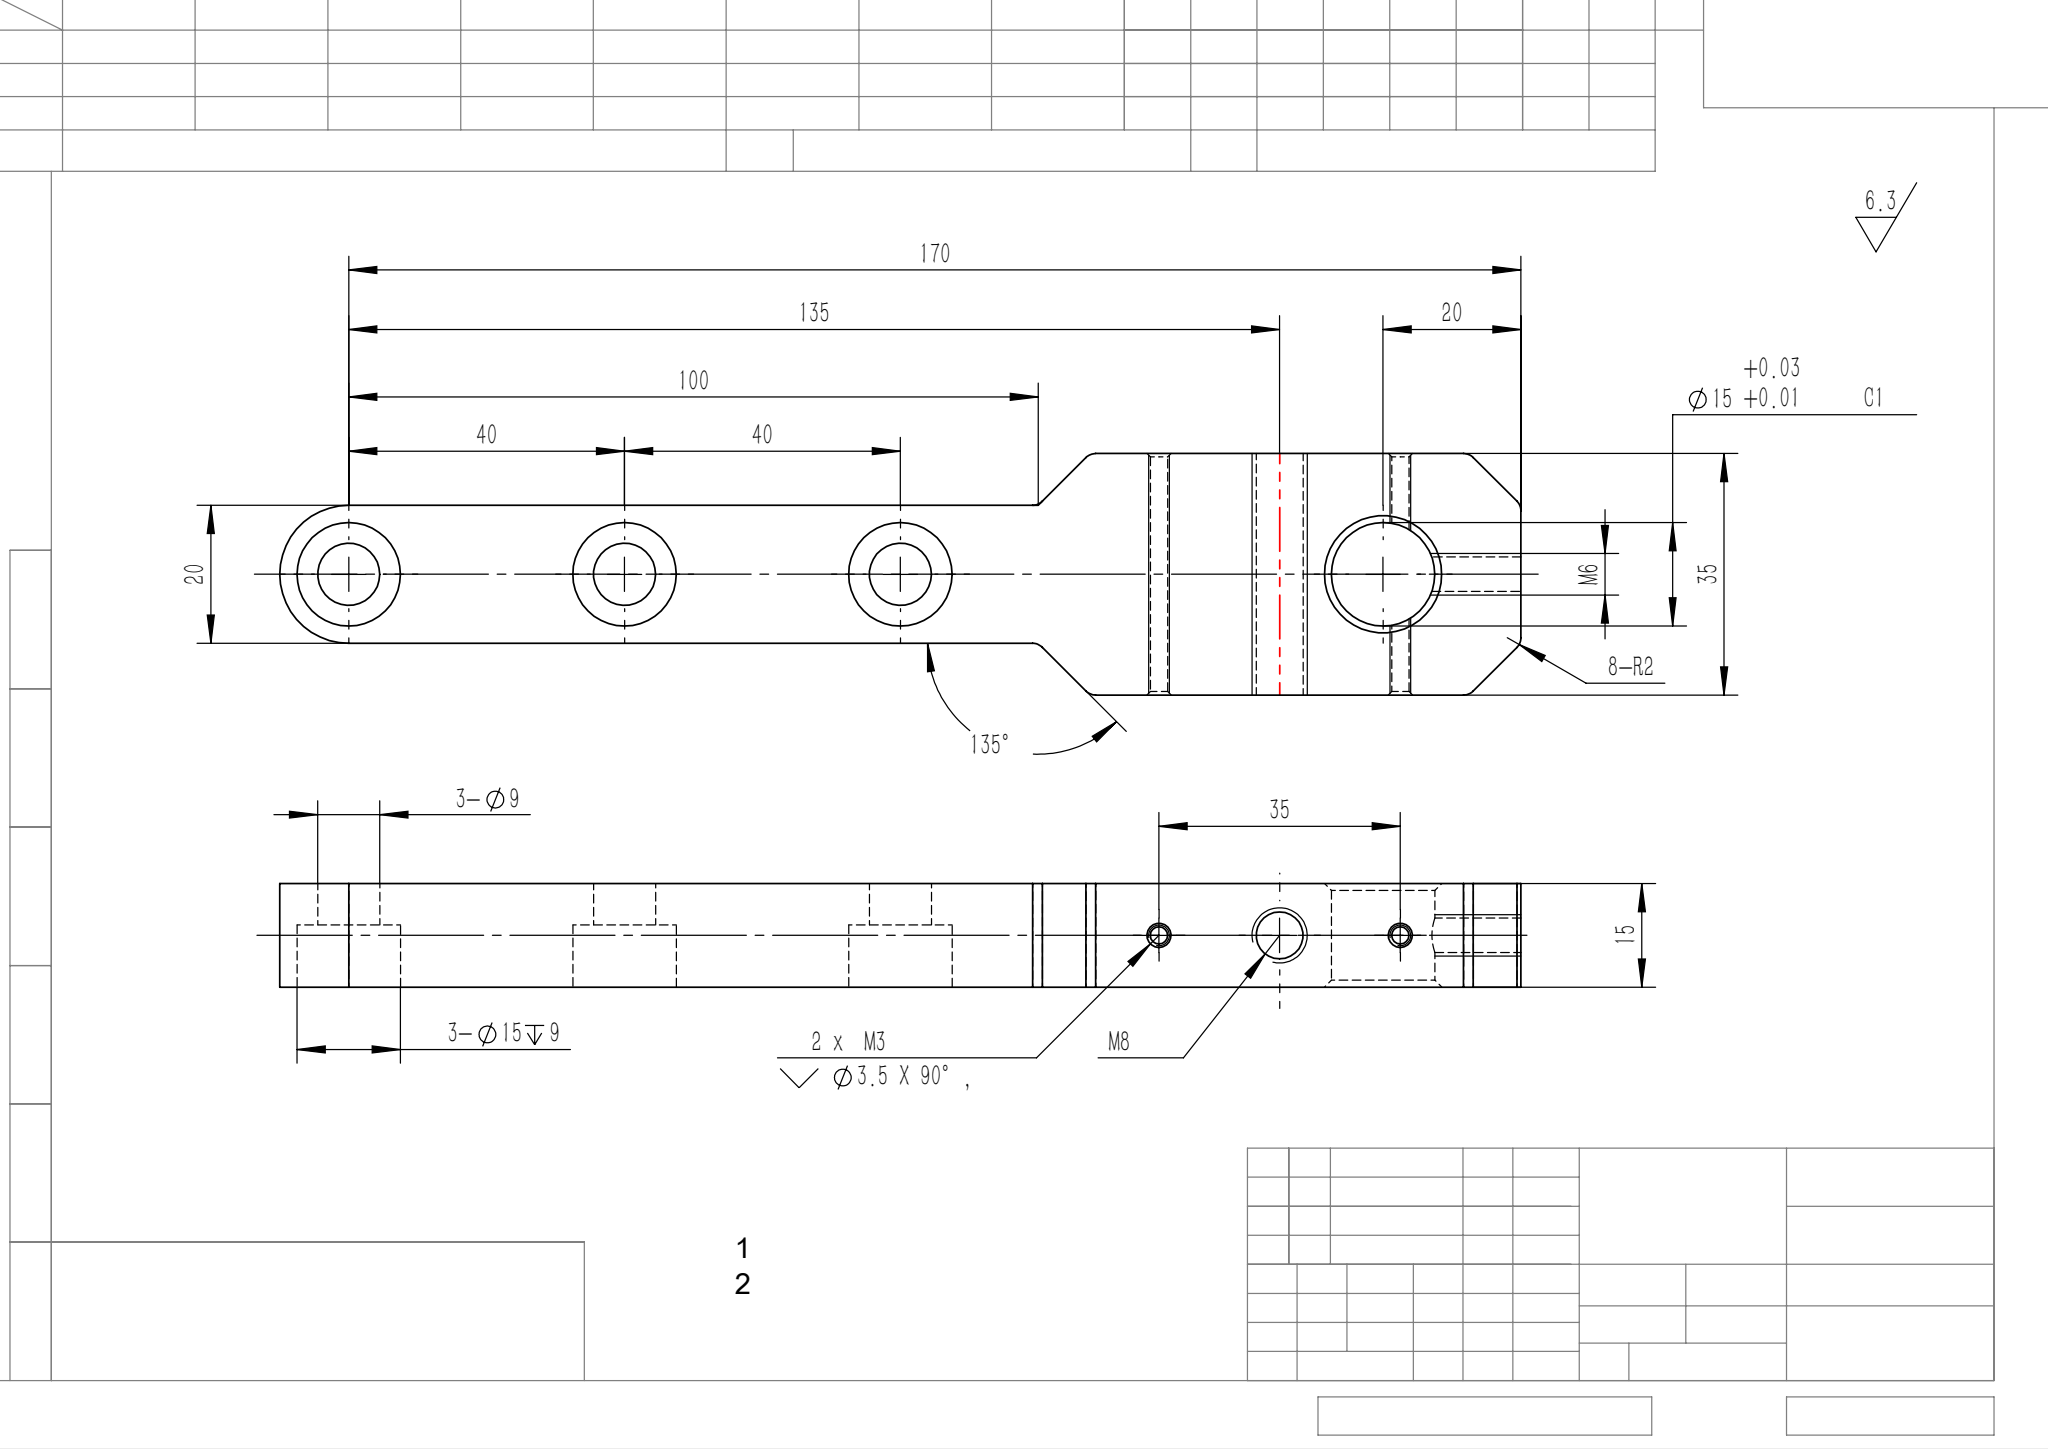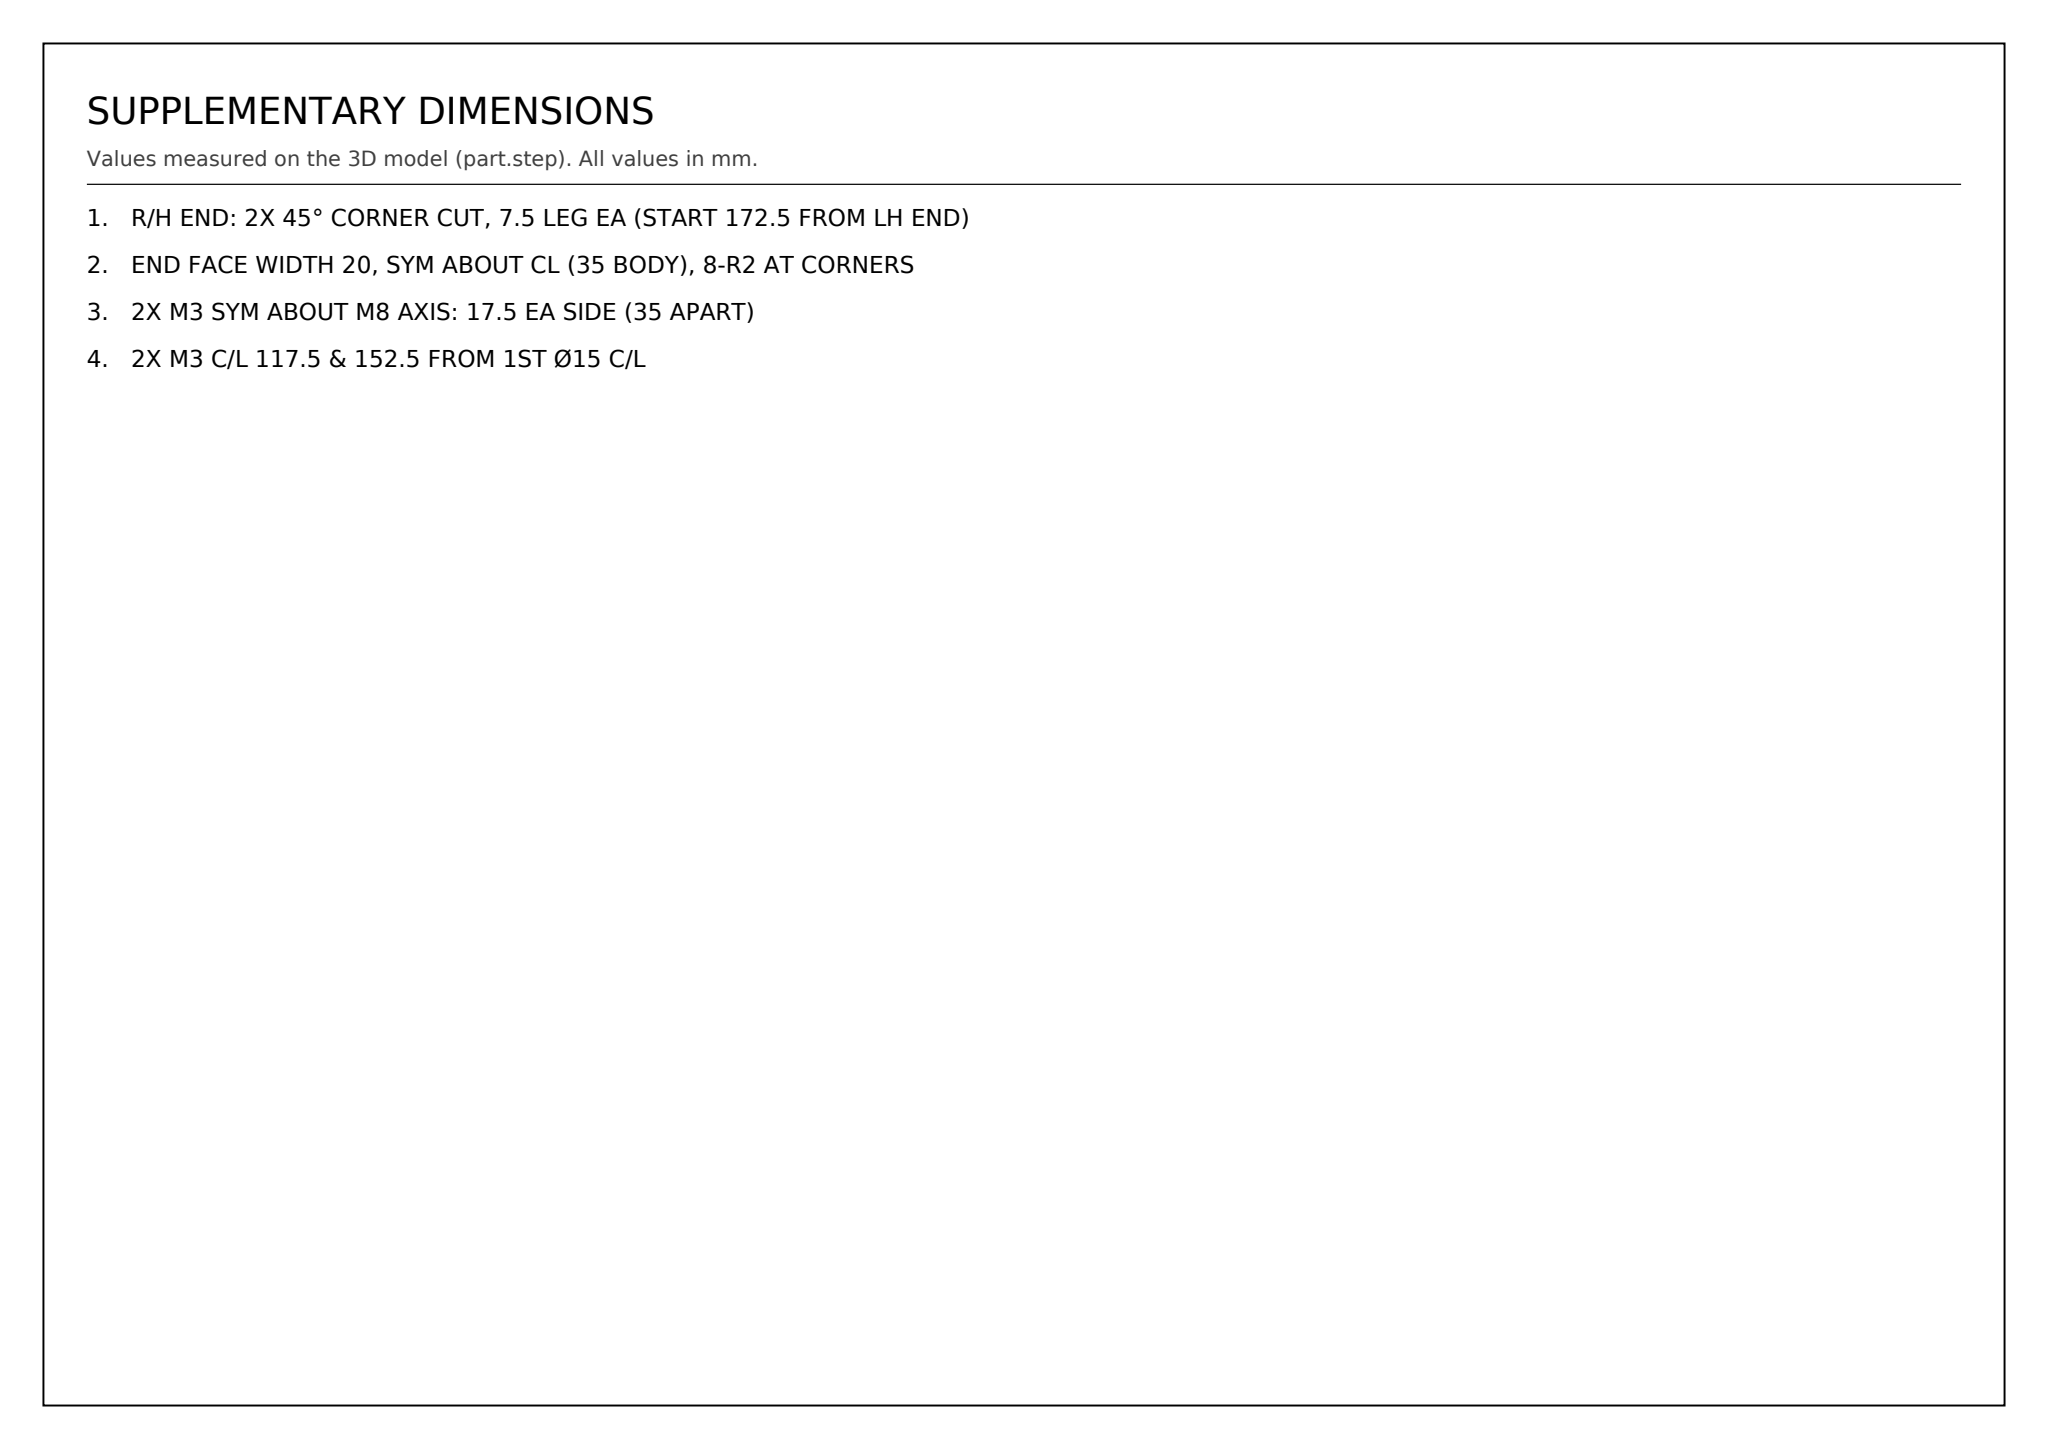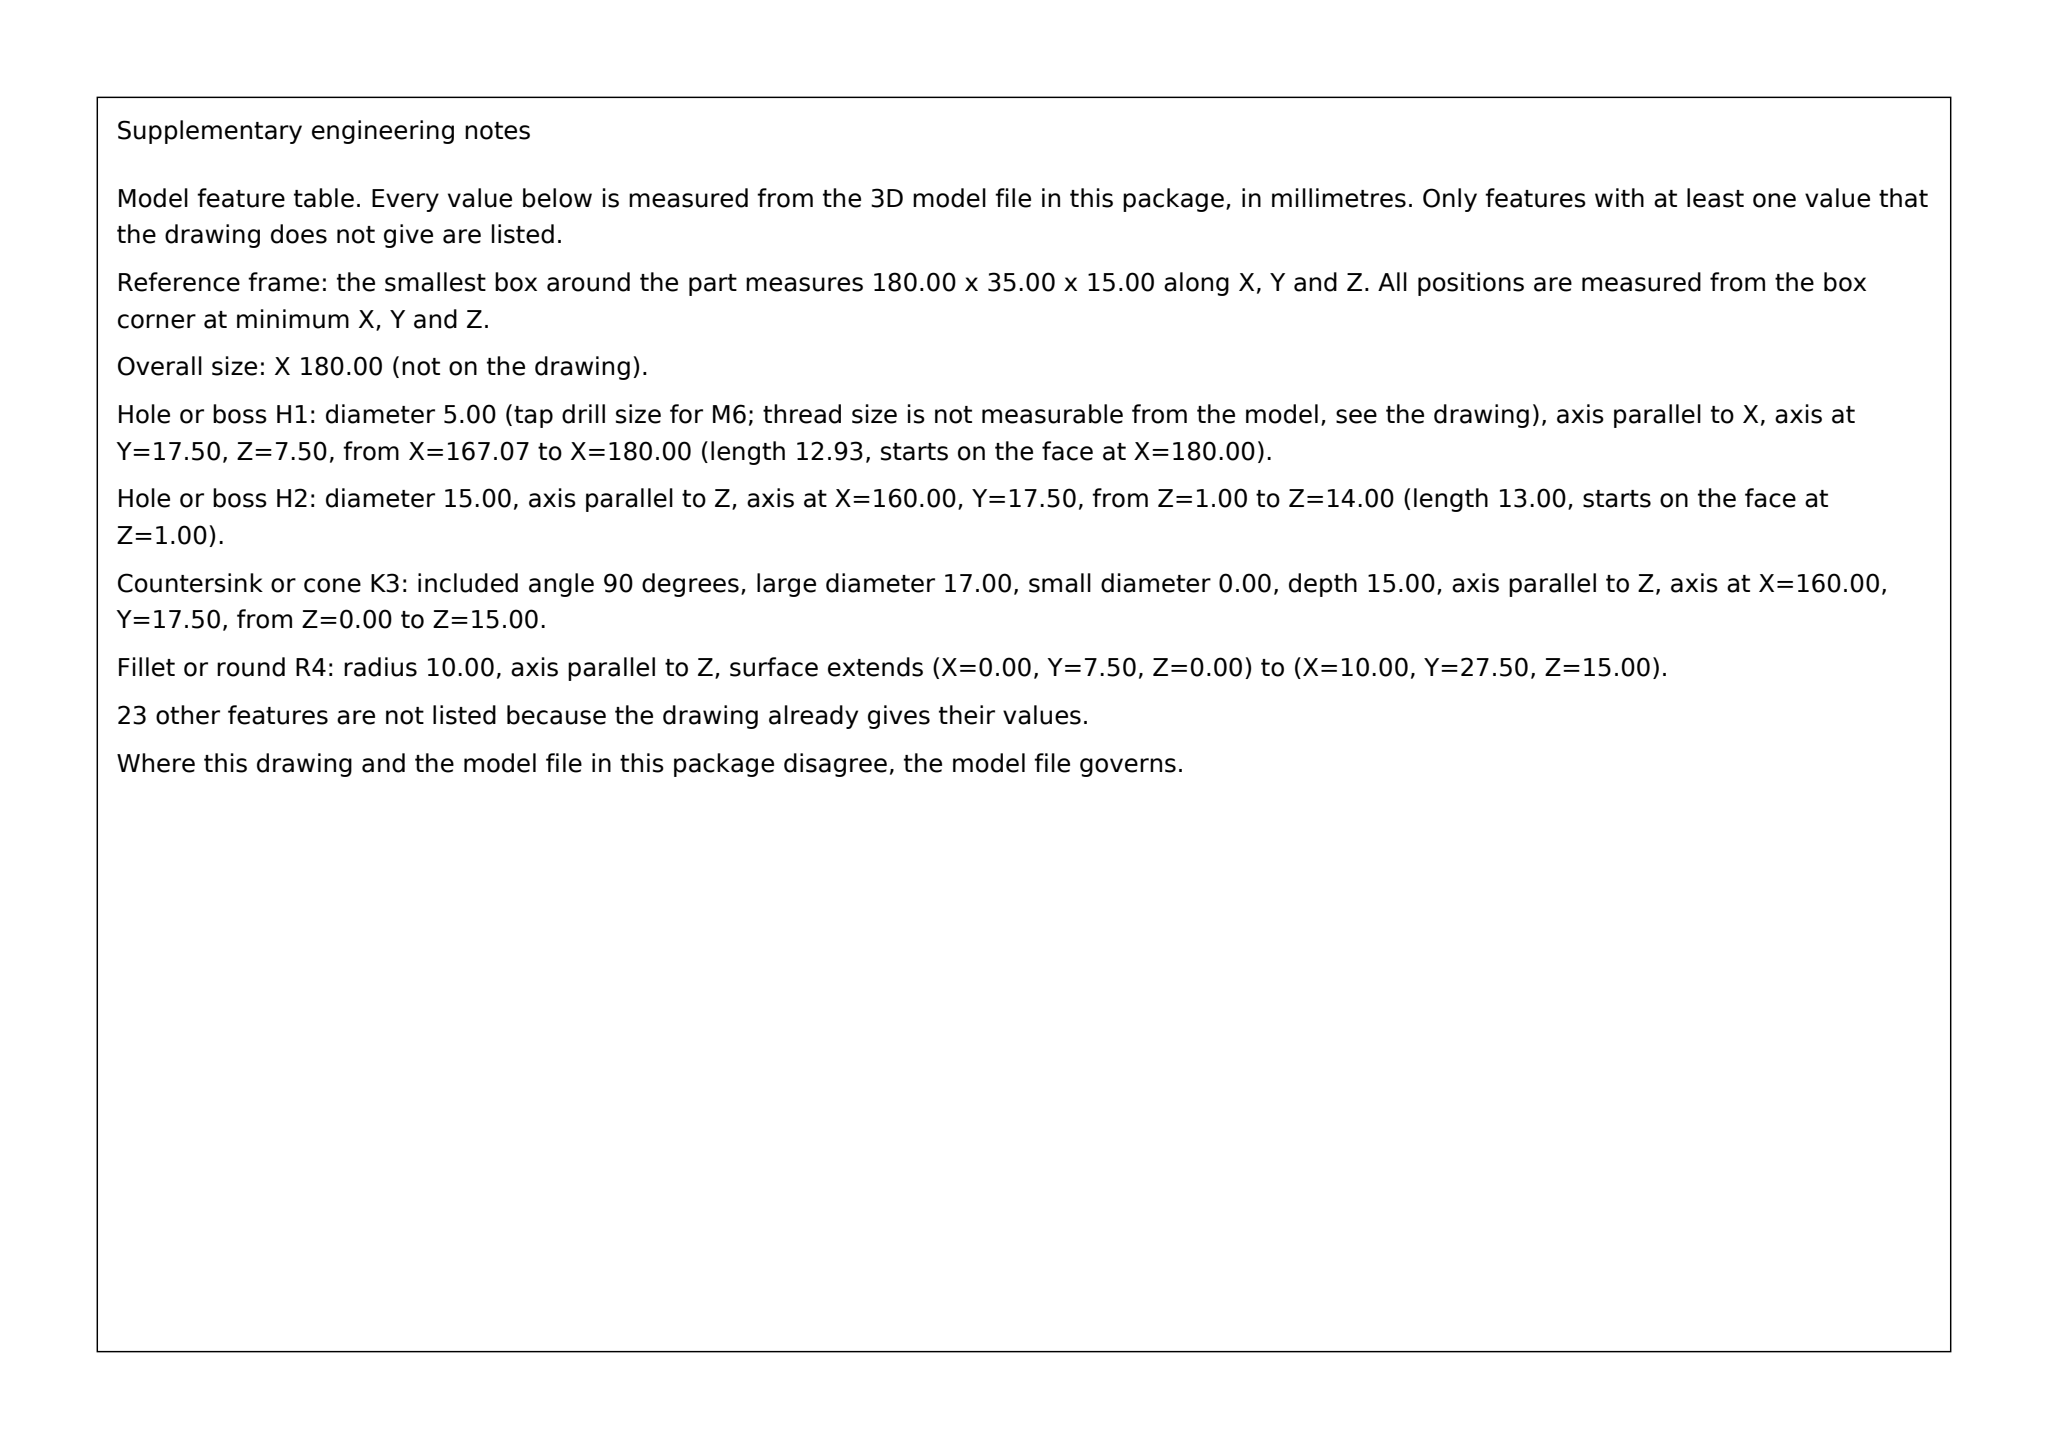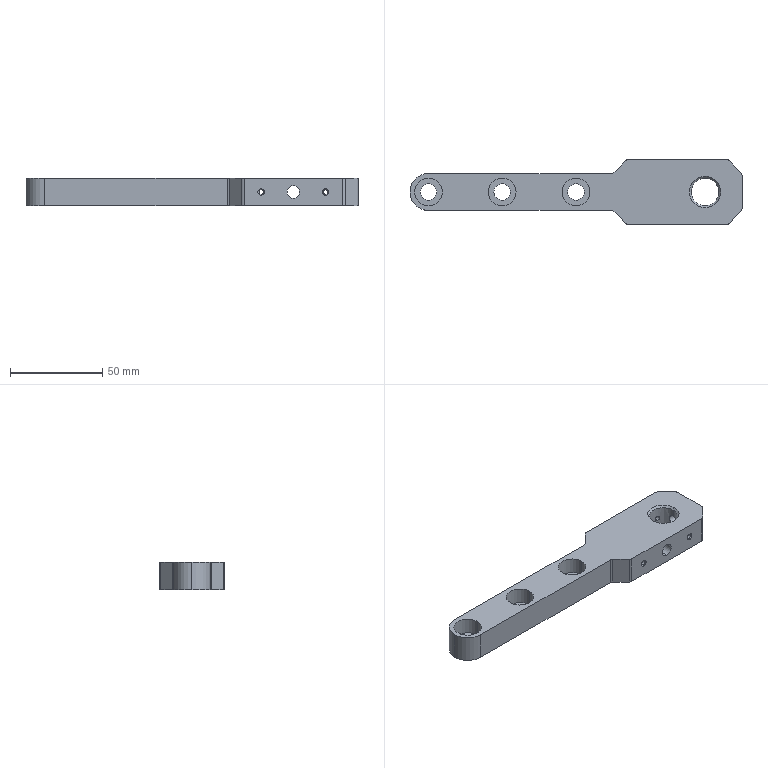Part | SolidWorks | mm | 1 solid | 60 faces | box 180 x 35 x 15 mm | volume 57000 mm3 | cylinder 34 | plane 14 | cone 12 | commonest cylinder face diameters 15 x8 4 x8 2.5 x6 9 x6 6.8 x2 5 x2 20 x2
Drawing notes:
R/H END: 2X 45° CORNER CUT, 7.5 LEG EA (START 172.5 FROM LH END) | from the solid: End face plane x=180 with y-planes 7.5 & 27.5; R2 fillet centers (171.67,33) & (178,8.33) fit 45° line x+y=207.5 / x-y=172.5 from (172.5,35)/(172.5,0)
END FACE WIDTH 20, SYM ABOUT CL (35 BODY), 8-R2 AT CORNERS | from the solid: axis_planes y=7.5 and y=27.5 bound end face at x=180; bbox y=35; Ø4 z-cylinders = R2 fillets at 4 corners
2X M3 SYM ABOUT M8 AXIS: 17.5 EA SIDE (35 APART) | from the solid: Ø2.5 Y-axis holes at x=127.5 & 162.5; M8 Ø6.8 hole at x=145
2X M3 C/L 117.5 & 152.5 FROM 1ST Ø15 C/L | from the solid: first Ø15 bore at x=10; M3 holes at x=127.5 and x=162.5